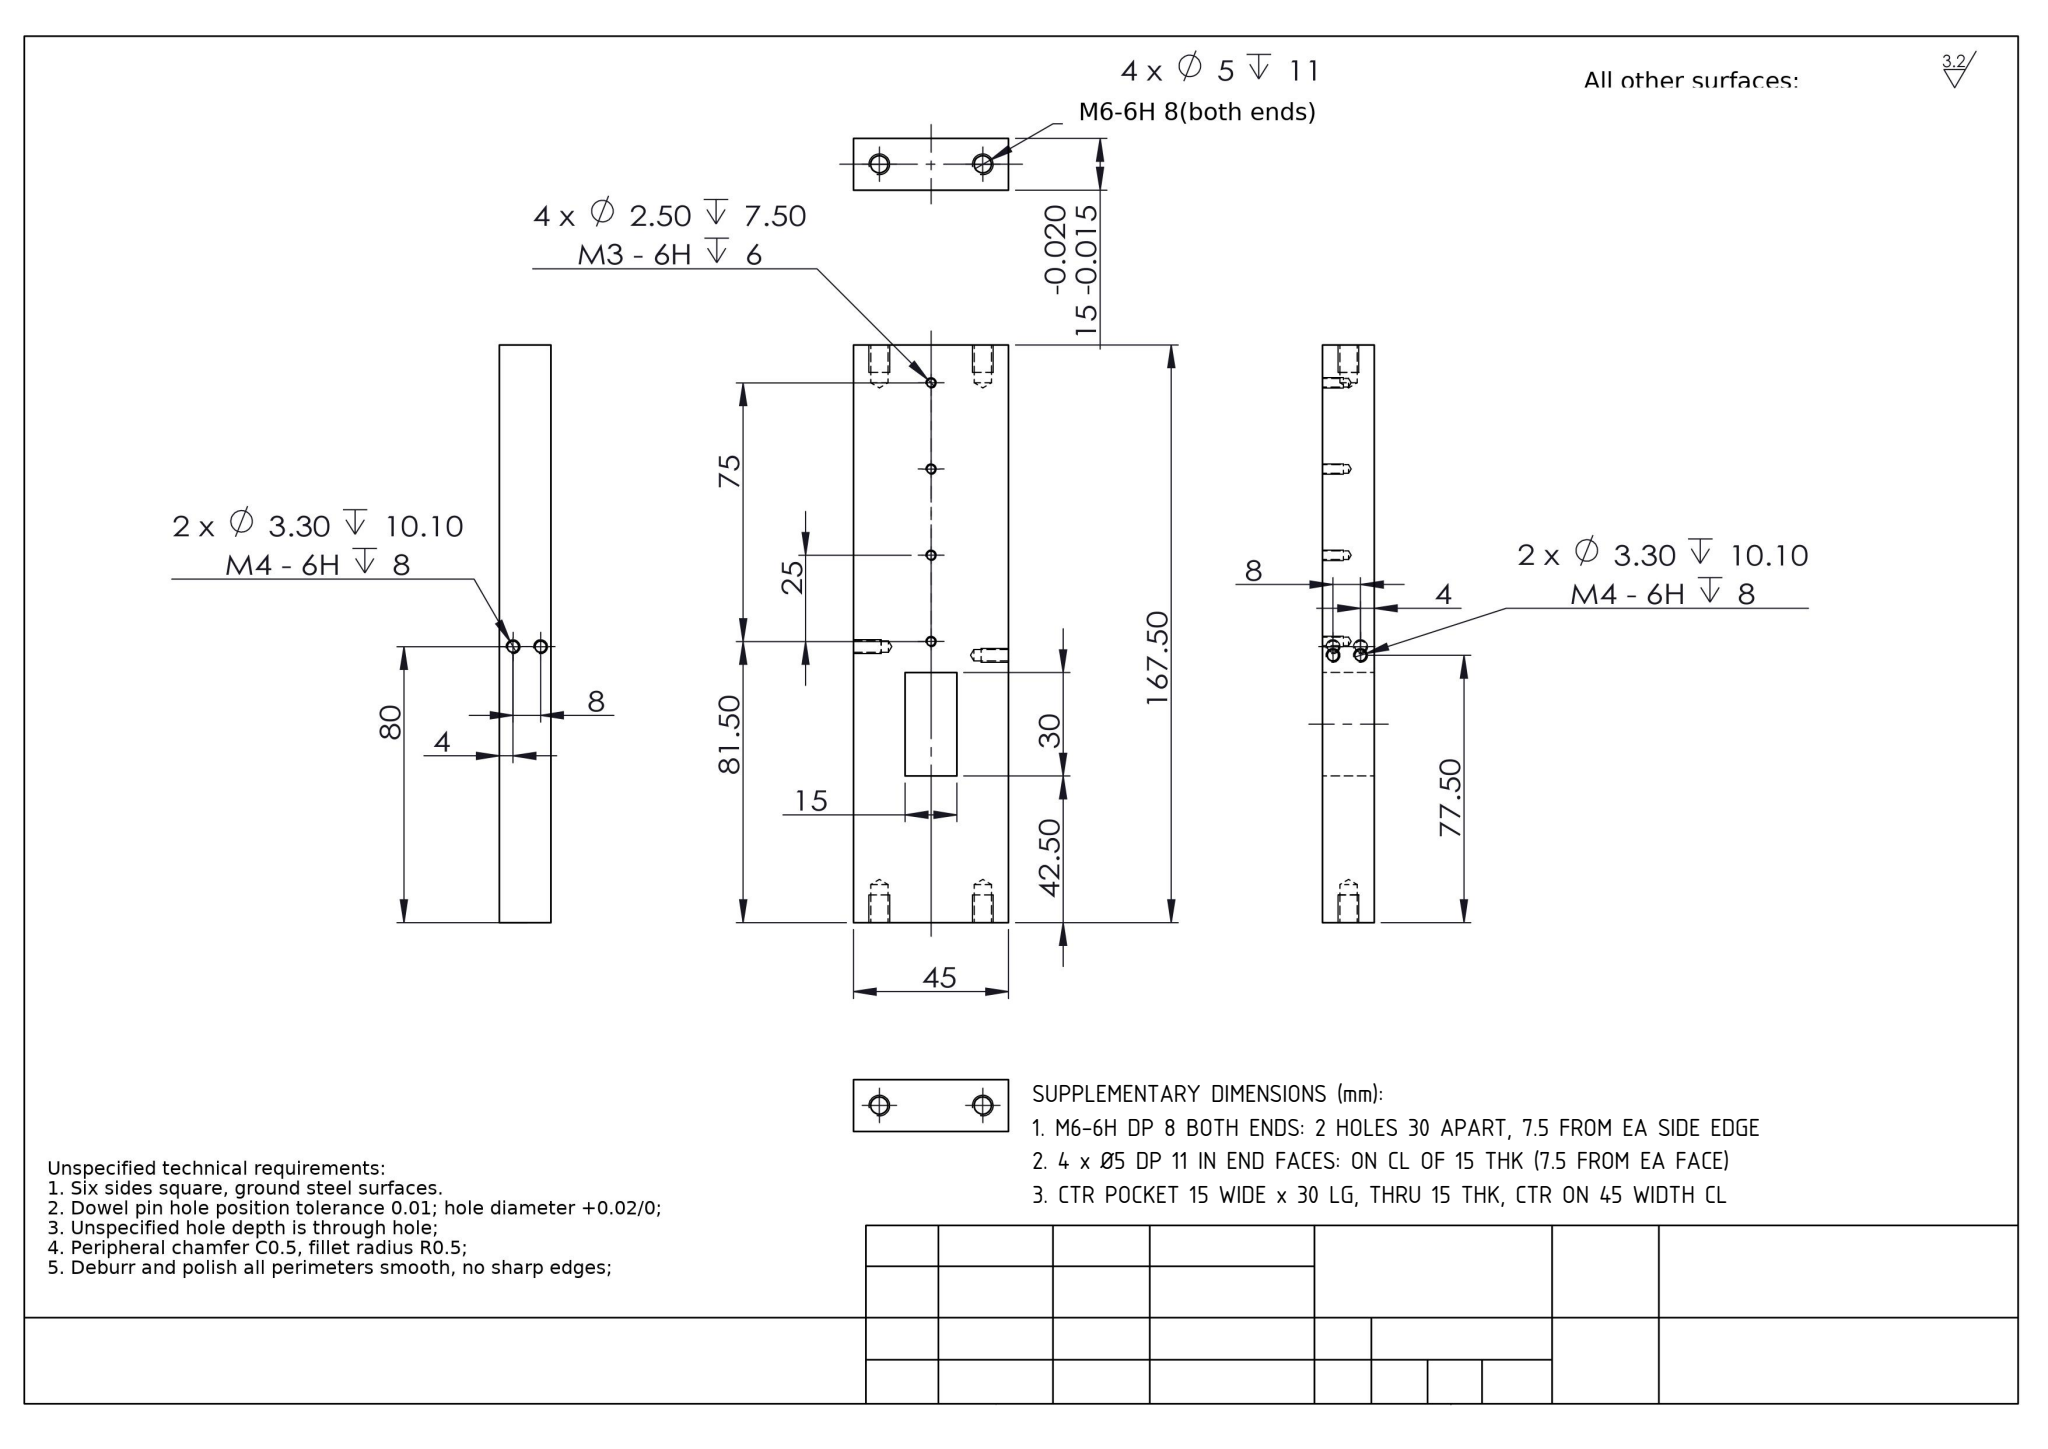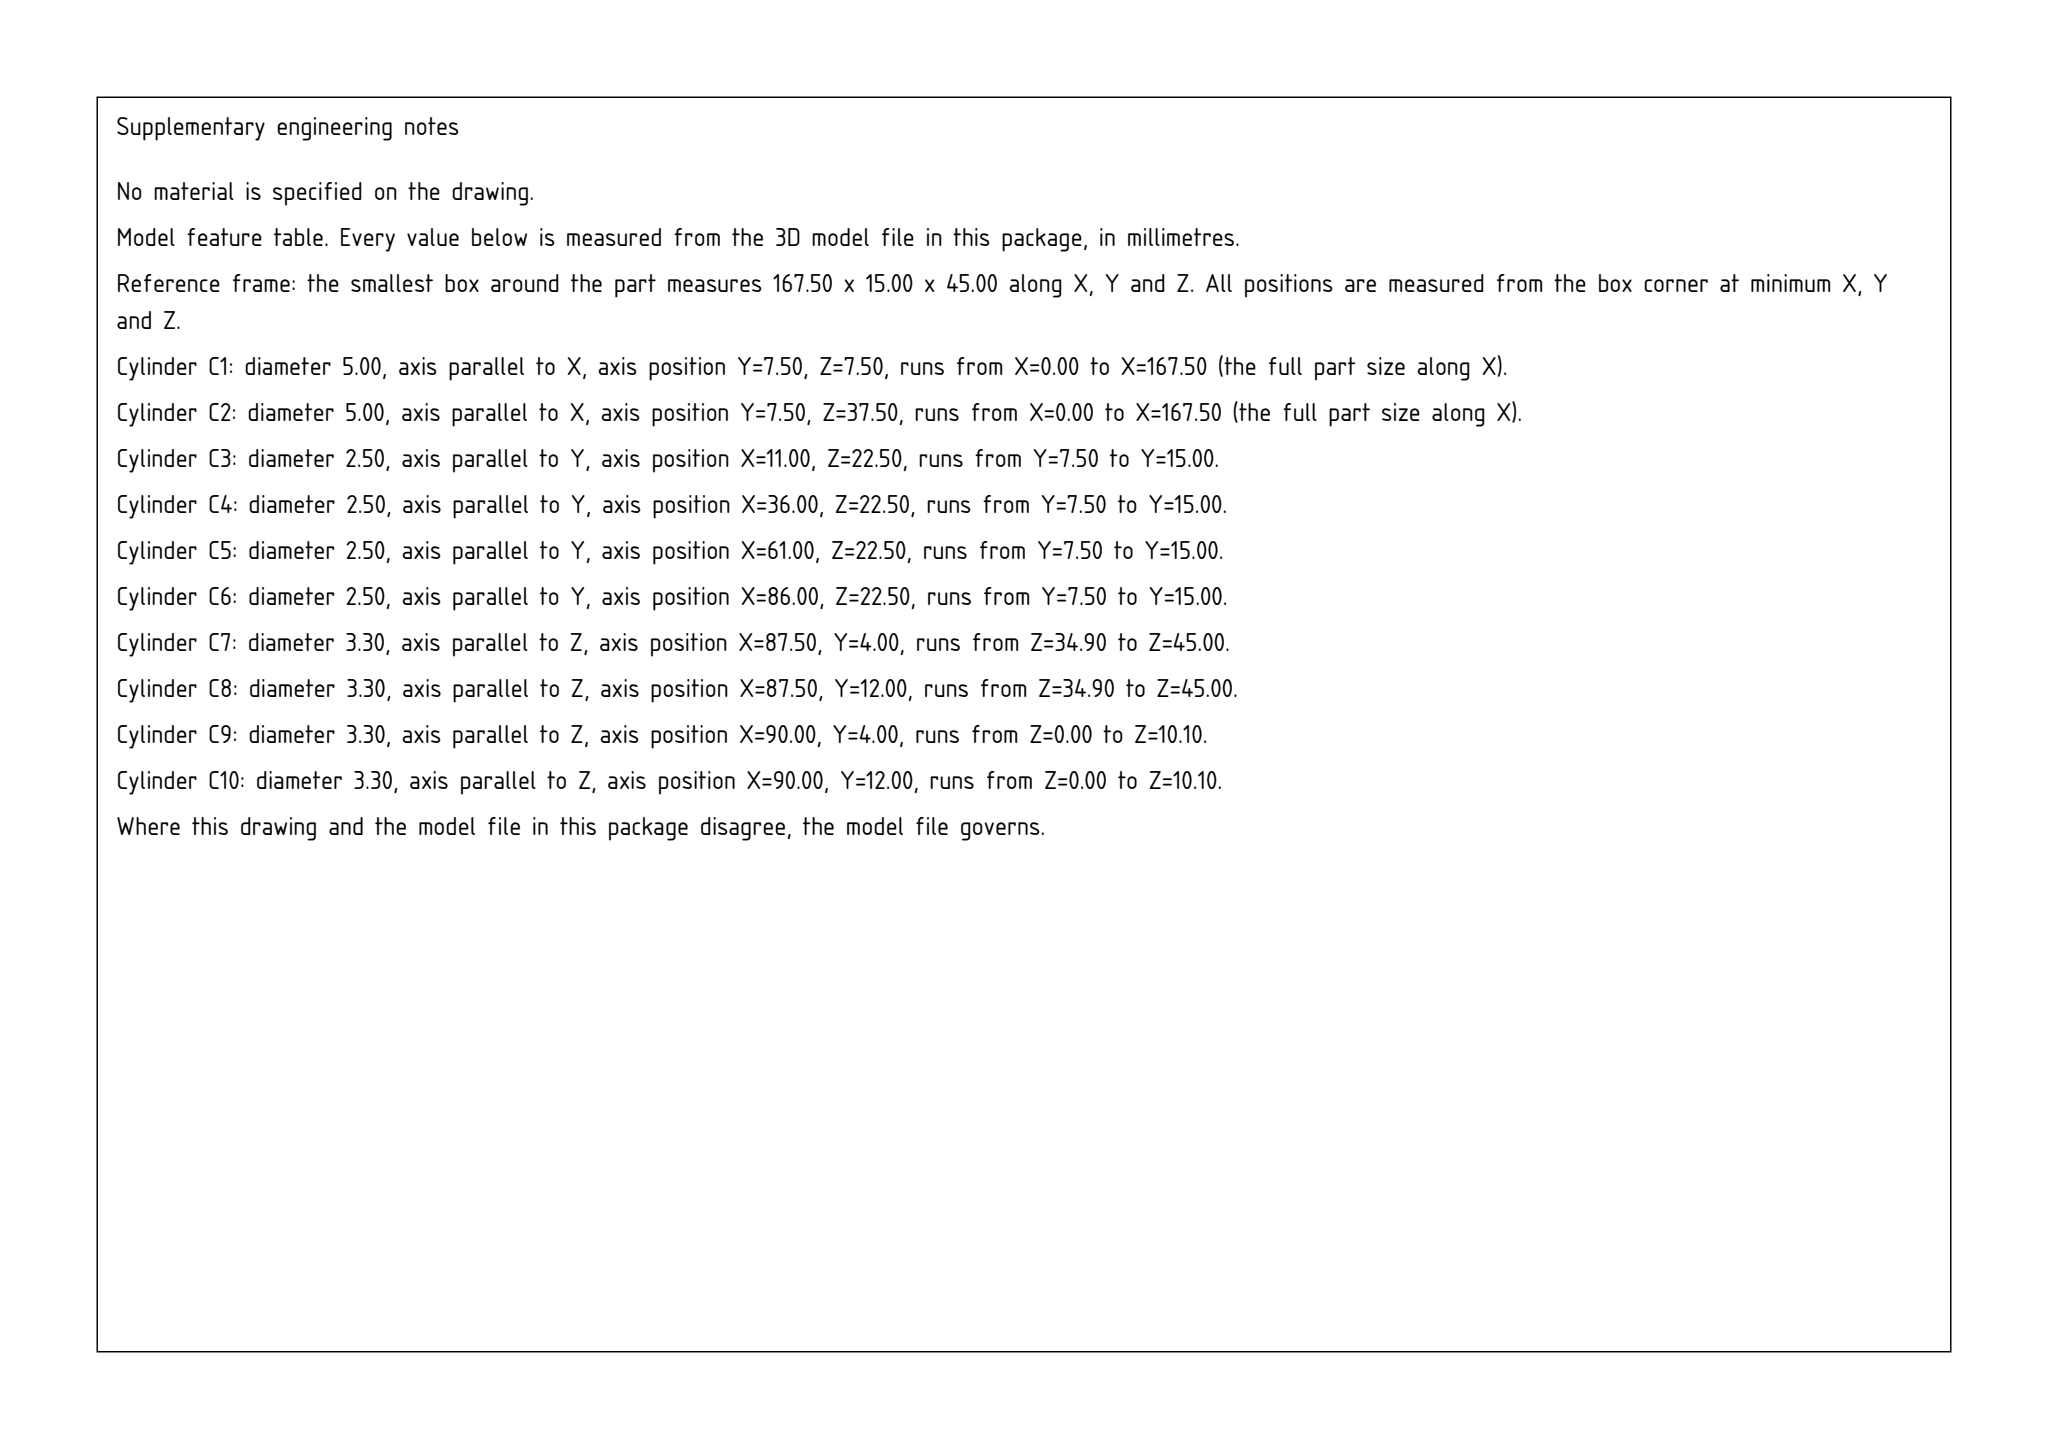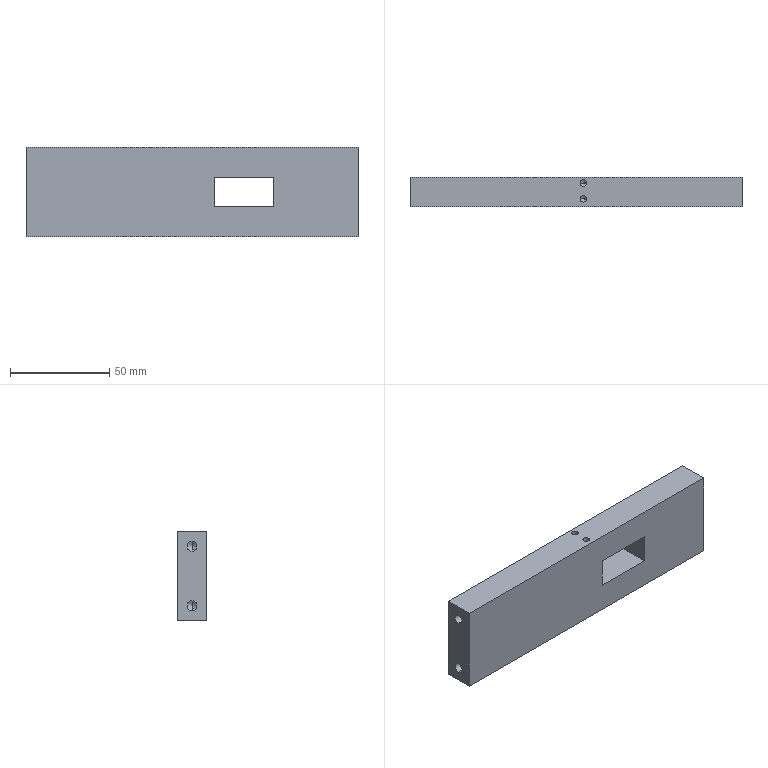Part | SolidWorks | mm | 1 solid | 58 faces | box 167.5 x 15 x 45 mm | volume 104900 mm3 | cylinder 24 | cone 24 | plane 10 | commonest cylinder face diameters 5 x8 2.5 x8 3.3 x8
build123d program:
from build123d import *

# Parameters (mm, degrees)
SKETCH1_W                  = 167.5
SKETCH1_H                  = 45
BOSS_EXTRUDE1_DEPTH        = 15
M6_TAPPED_HOLE1_AT_2_COUNT = 2
M6_TAPPED_HOLE1_AT_2_PITCH = 30
SKETCH6_W                  = 30
SKETCH6_H                  = 15
CUT_EXTRUDE1_DEPTH         = 89.007
M4_TAPPED_HOLE1_D          = 3.3
M4_TAPPED_HOLE1_DEPTH      = 10.1
M4_TAPPED_HOLE1_TIP        = 0.9914
M4_TAPPED_HOLE2_D          = 3.3
M4_TAPPED_HOLE2_DEPTH      = 10.1
M4_TAPPED_HOLE2_TIP        = 0.9914
LPATTERN2_COUNT            = 4
LPATTERN2_PITCH            = 25


with BuildPart() as part:
    # Sketch1 → Boss-Extrude1 (new body)
    with BuildSketch(Plane(origin=(0, 0, 0), x_dir=(1, 0, 0), z_dir=(0, 1, 0))):
        Rectangle(SKETCH1_W, SKETCH1_H)
    extrude(amount=BOSS_EXTRUDE1_DEPTH)

    # Sketch3 → M3 Tapped Hole1 (revolve, cut)
    with BuildSketch(Plane(origin=(-72.75, 15, 0), x_dir=(0, 0, 1), z_dir=(1, 0, 0))):
        Polygon((0, 0), (0, 8.251), (1.25, 7.5), (1.25, 0), align=None)
    m3_tapped_hole1 = revolve(axis=Axis((-72.75, 21.35, 0), (0, -1, 0)), mode=Mode.SUBTRACT)

    # Sketch5 → M6 Tapped Hole1 (revolve, cut)
    with BuildSketch(Plane(origin=(83.75, 7.5, -15), x_dir=(0, 0, -1), z_dir=(0, 1, 0))):
        Polygon((0, 0), (0, 12.502), (2.5, 11), (2.5, 0), align=None)
    m6_tapped_hole1 = revolve(axis=Axis((90.1, 7.5, -15), (-1, 0, 0)), mode=Mode.SUBTRACT)

    # M6 Tapped Hole1 at 2: M6 Tapped Hole1 ×2
    with Locations(*[(0, 0, i * M6_TAPPED_HOLE1_AT_2_PITCH) for i in range(1, M6_TAPPED_HOLE1_AT_2_COUNT)]):
        add(m6_tapped_hole1, mode=Mode.SUBTRACT)

    # Sketch6 → Cut-Extrude1 (cut, through all)
    with BuildSketch(Plane.XZ):
        with Locations((26.25, 0)):
            Rectangle(SKETCH6_W, SKETCH6_H)
    extrude(amount=-CUT_EXTRUDE1_DEPTH, mode=Mode.SUBTRACT)

    # M4 Tapped Hole1
    with Locations(Plane.XY.offset(22.5)):
        with Locations((3.75, 4), (3.75, 12)):
            Hole(M4_TAPPED_HOLE1_D / 2, depth=M4_TAPPED_HOLE1_DEPTH)
            with Locations((0, 0, -(M4_TAPPED_HOLE1_DEPTH + M4_TAPPED_HOLE1_TIP / 2))):  # 118° drill point
                Cone(0, M4_TAPPED_HOLE1_D / 2, M4_TAPPED_HOLE1_TIP, mode=Mode.SUBTRACT)

    # M4 Tapped Hole2
    with Locations(Plane(origin=(0, 0, -22.5), x_dir=(-1, 0, 0), z_dir=(0, 0, -1))):
        with Locations((-6.25, 4), (-6.25, 12)):
            Hole(M4_TAPPED_HOLE2_D / 2, depth=M4_TAPPED_HOLE2_DEPTH)
            with Locations((0, 0, -(M4_TAPPED_HOLE2_DEPTH + M4_TAPPED_HOLE2_TIP / 2))):  # 118° drill point
                Cone(0, M4_TAPPED_HOLE2_D / 2, M4_TAPPED_HOLE2_TIP, mode=Mode.SUBTRACT)

    # LPattern2: M3 Tapped Hole1 ×4
    with Locations(*[(i * LPATTERN2_PITCH, 0, 0) for i in range(1, LPATTERN2_COUNT)]):
        add(m3_tapped_hole1, mode=Mode.SUBTRACT)

    # Mirror1: M6 Tapped Hole1 across plane
    add(m6_tapped_hole1.mirror(Plane(origin=(0, 0, 0), x_dir=(0, 0, 1), z_dir=(1, 0, 0))), mode=Mode.SUBTRACT)

    # Mirror1 copy 1 sketch → Mirror1 copy 1 (revolve, cut)
    with BuildSketch(Plane(origin=(-83.75, 7.5, 15), x_dir=(0, 0, -1), z_dir=(0, 1, 0))):
        Polygon((0, 0), (0, -12.502), (2.5, -11), (2.5, 0), align=None)
    revolve(axis=Axis((-90.1, 7.5, 15), (-1, 0, 0)), mode=Mode.SUBTRACT)


solid = part.part